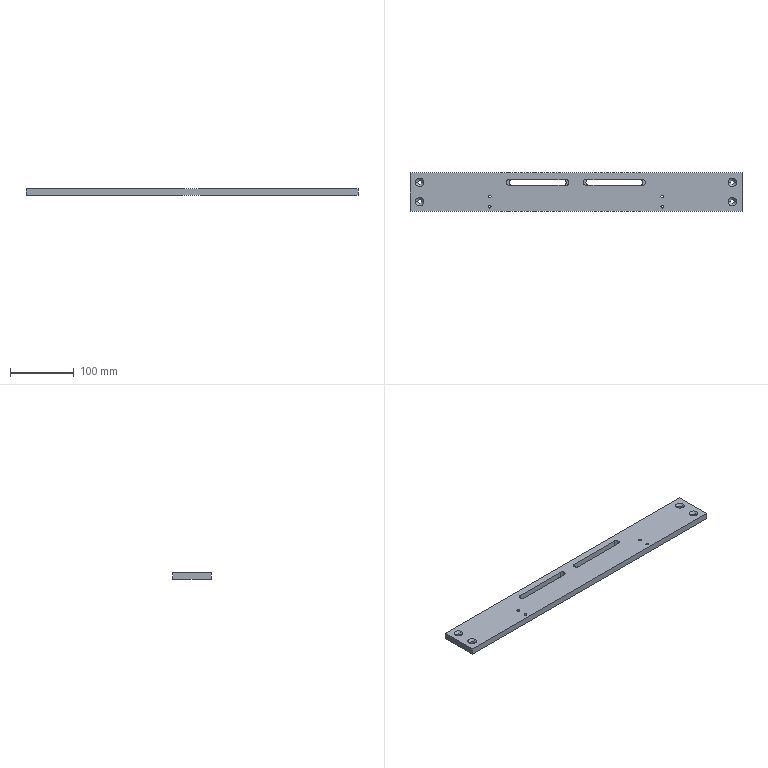Component | SolidWorks | GuideWheelAdjustingPlate2-1 | 1 solid | 50 faces | box 520 x 60 x 10 mm | volume 292402 mm3 | cylinder 28 | plane 14 | cone 8 | commonest cylinder face diameters 9 x12 6.5 x8 4.2 x8
build123d program:
from build123d import *

# Parameters (mm, degrees)
SKETCH1_2_W                                          = 520
SKETCH1_2_H                                          = 30
BOSS_EXTRUDE1_DEPTH                                  = 10
CUT_EXTRUDE1_DEPTH                                   = 261.624
SKETCH3_W                                            = 520
SKETCH3_H                                            = 10
BOSS_EXTRUDE2_DEPTH                                  = 30
M5_TAPPED_HOLE1_D                                    = 4.2
COUNTERSUNK_HOLE_1_FOR_M6_HEX_SOCKET_COU_D           = 6.5
COUNTERSUNK_HOLE_1_FOR_M6_HEX_SOCKET_COU_CSINK_D     = 13.44
COUNTERSUNK_HOLE_1_FOR_M6_HEX_SOCKET_COU_CSINK_ANGLE = 90
SLOTENDRELIEF_DEPTH                                  = 8.5


with BuildPart() as part:
    # Sketch1_2 → Boss-Extrude1 (new body)
    with BuildSketch(Plane.XY):
        Rectangle(SKETCH1_2_W, SKETCH1_2_H)
    extrude(amount=BOSS_EXTRUDE1_DEPTH)

    # Sketch2 → Cut-Extrude1 (cut, through all)
    with BuildSketch(Plane.XY.offset(10)):
        with BuildLine():
            Line((-100, 4.5), (-20, 4.5))
            ThreePointArc((-20, 4.5), (-15.5, 0), (-20, -4.5))
            Line((-20, -4.5), (-100, -4.5))
            ThreePointArc((-100, -4.5), (-104.5, 0), (-100, 4.5))
        make_face()
        with BuildLine():
            Line((100, 4.5), (20, 4.5))
            ThreePointArc((20, 4.5), (15.5, 0), (20, -4.5))
            Line((20, -4.5), (100, -4.5))
            ThreePointArc((100, -4.5), (104.5, 0), (100, 4.5))
        make_face()
    extrude(amount=-CUT_EXTRUDE1_DEPTH, mode=Mode.SUBTRACT)

    # Sketch3 → Boss-Extrude2 (add)
    with BuildSketch(Plane.XZ.offset(15)):
        with Locations((0, 5)):
            Rectangle(SKETCH3_W, SKETCH3_H)
    extrude(amount=BOSS_EXTRUDE2_DEPTH)

    # M5 Tapped Hole1 (through all)
    with Locations(Plane.XY.offset(10)):
        with Locations((-135, -22), (-135, -38), (135, -22), (135, -38)):
            Hole(M5_TAPPED_HOLE1_D / 2)

    # Countersunk Hole 1 for M6 Hex Socket Cou (through all)
    with Locations(Plane.XY.offset(10)):
        with Locations((-245, 0), (-245, -30), (245, 0), (245, -30)):
            CounterSinkHole(COUNTERSUNK_HOLE_1_FOR_M6_HEX_SOCKET_COU_D / 2, COUNTERSUNK_HOLE_1_FOR_M6_HEX_SOCKET_COU_CSINK_D / 2, counter_sink_angle=COUNTERSUNK_HOLE_1_FOR_M6_HEX_SOCKET_COU_CSINK_ANGLE)

    # Sketch1 → SlotEndRelief (cut)
    with BuildSketch(Plane.XY.offset(10)):
        with BuildLine():
            Line((-100, 4.5), (-104.5, 4.5))
            ThreePointArc((-104.5, 4.5), (-109, 0), (-104.5, -4.5))
            Line((-104.5, -4.5), (-100, -4.5))
            Line((-100, -4.5), (-100, 4.5))
        make_face()
        with BuildLine():
            Line((-20, 4.5), (-15.5, 4.5))
            ThreePointArc((-15.5, 4.5), (-11, 0), (-15.5, -4.5))
            Line((-15.5, -4.5), (-20, -4.5))
            Line((-20, -4.5), (-20, 4.5))
        make_face()
        with BuildLine():
            Line((20, 4.5), (15.5, 4.5))
            ThreePointArc((15.5, 4.5), (11, 0), (15.5, -4.5))
            Line((15.5, -4.5), (20, -4.5))
            Line((20, -4.5), (20, 4.5))
        make_face()
        with BuildLine():
            Line((100, 4.5), (104.5, 4.5))
            ThreePointArc((104.5, 4.5), (109, 0), (104.5, -4.5))
            Line((104.5, -4.5), (100, -4.5))
            Line((100, -4.5), (100, 4.5))
        make_face()
    extrude(amount=-SLOTENDRELIEF_DEPTH, mode=Mode.SUBTRACT)


solid = part.part

# Placed as in the assembly
solid = solid.moved(Location((-394.97, -205, 0), (0, 0, 0)))